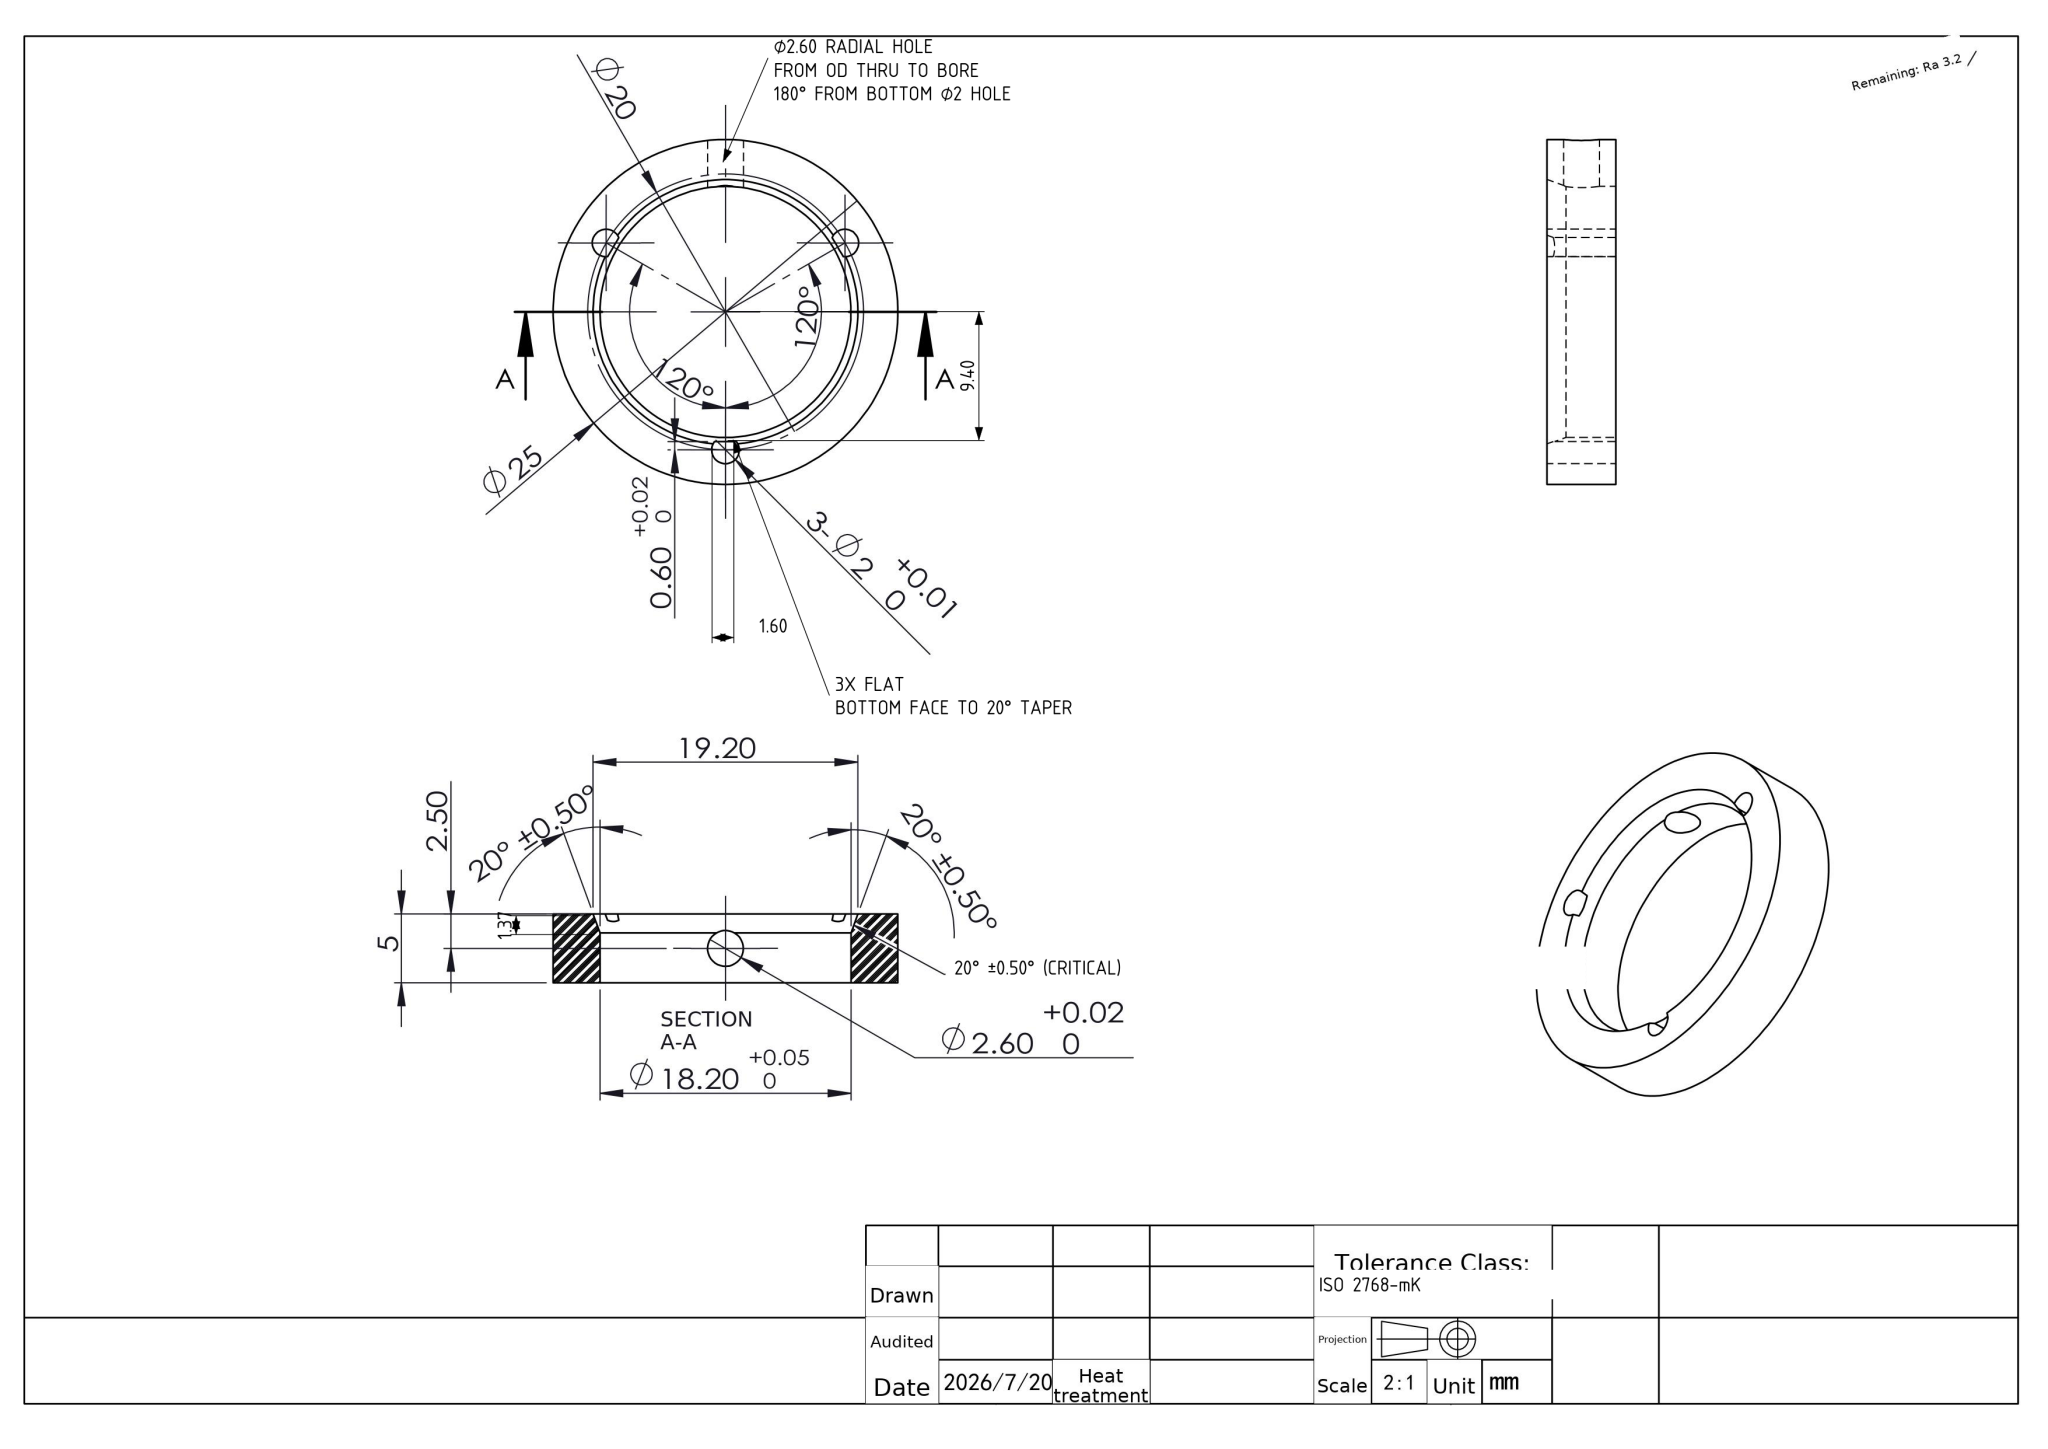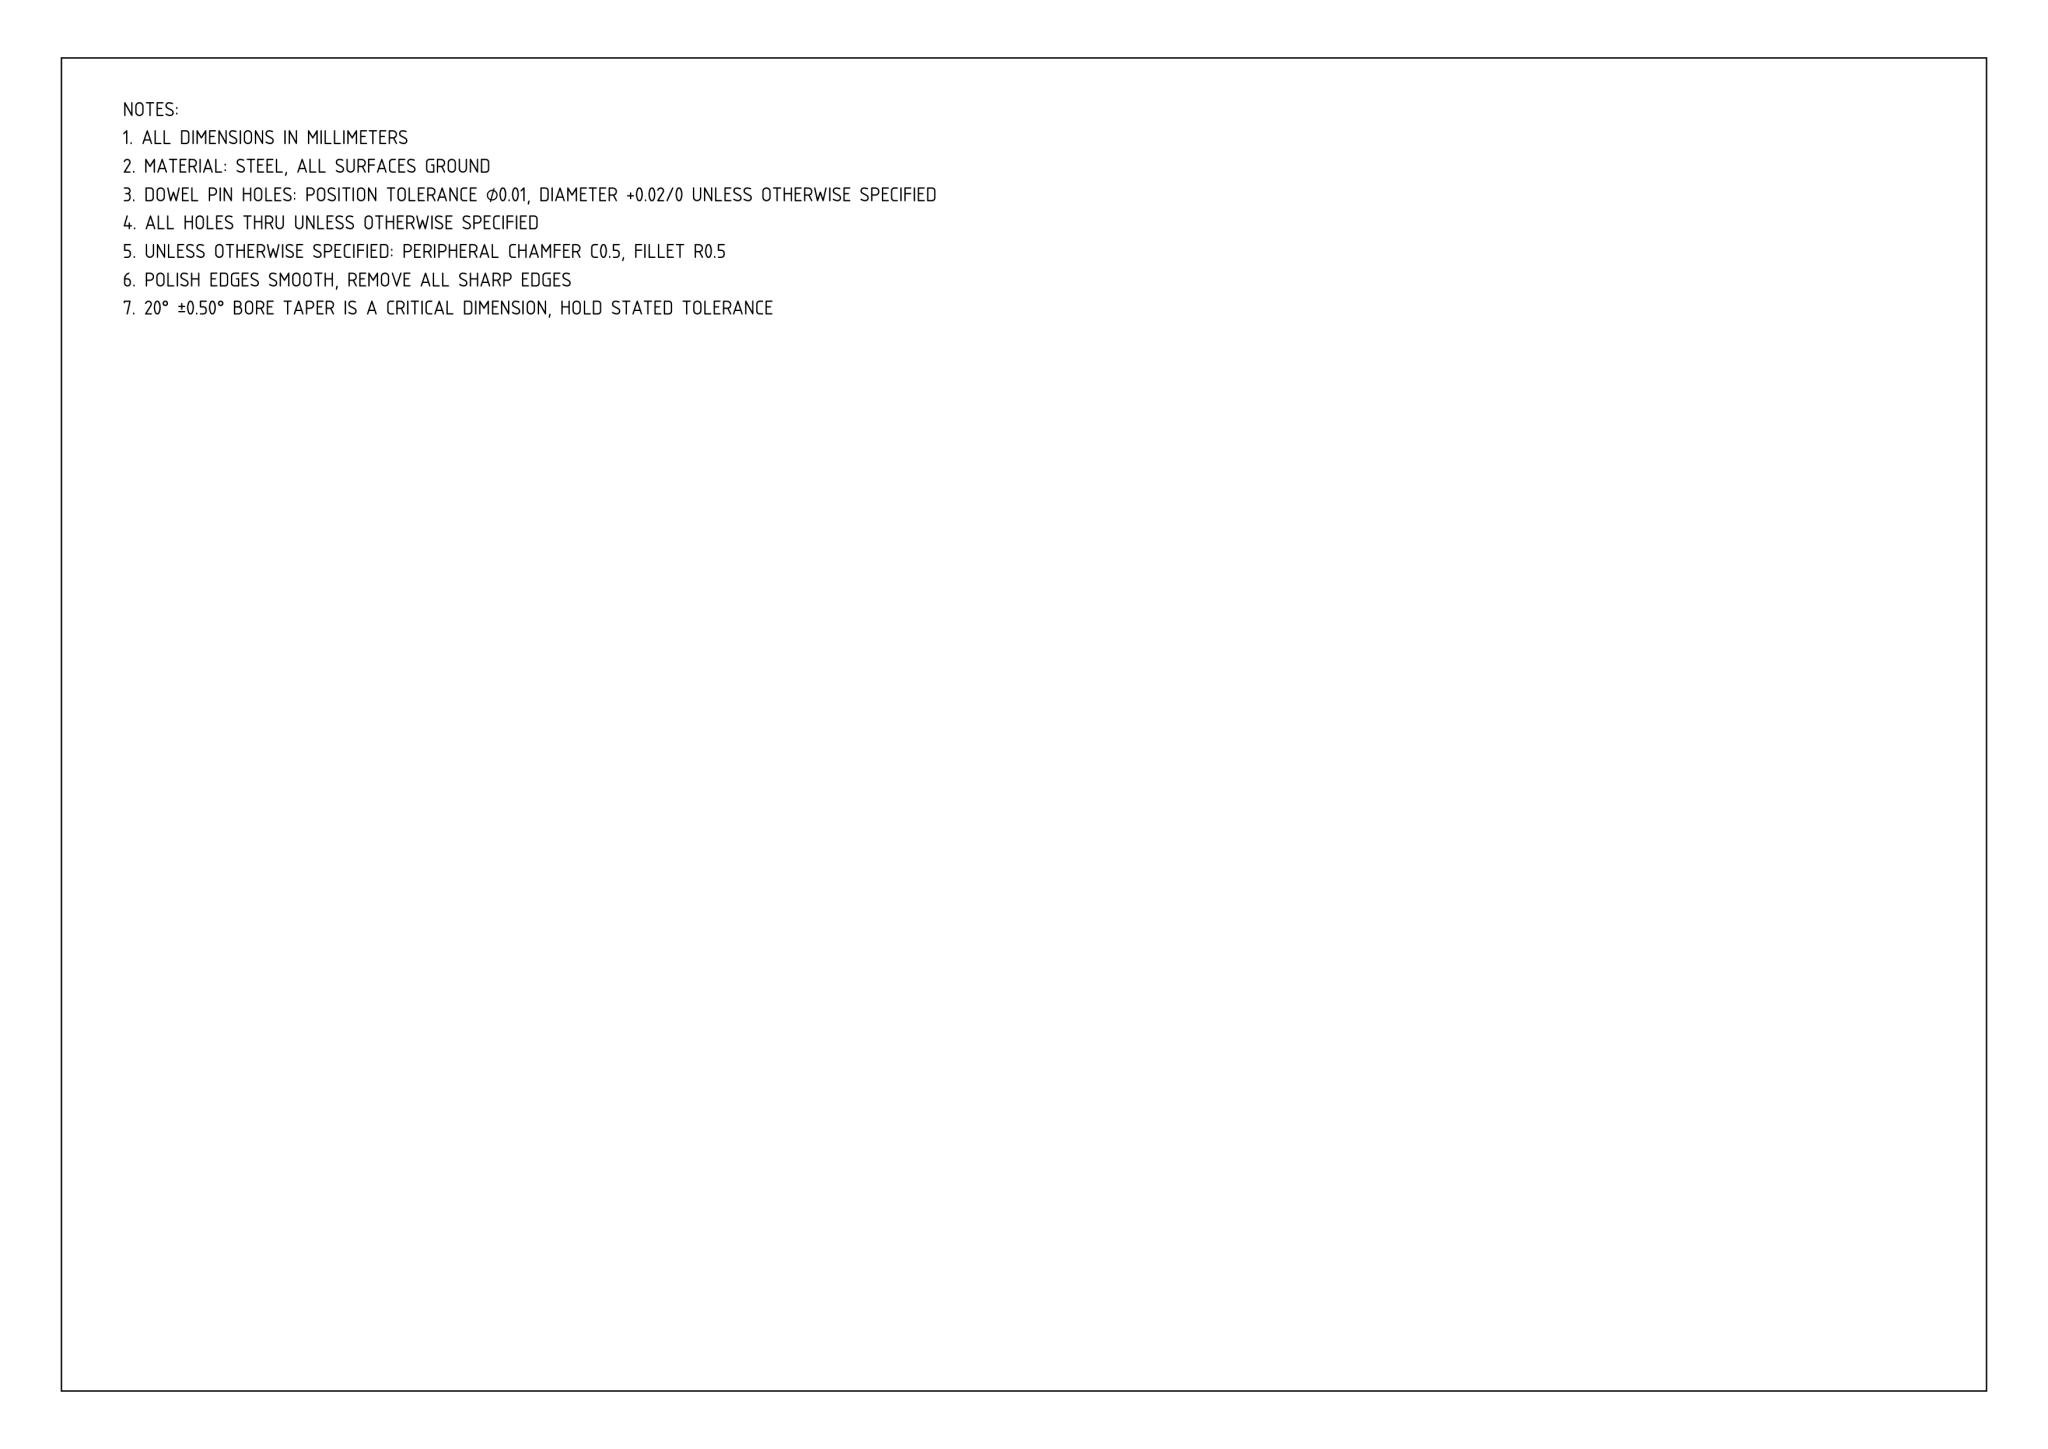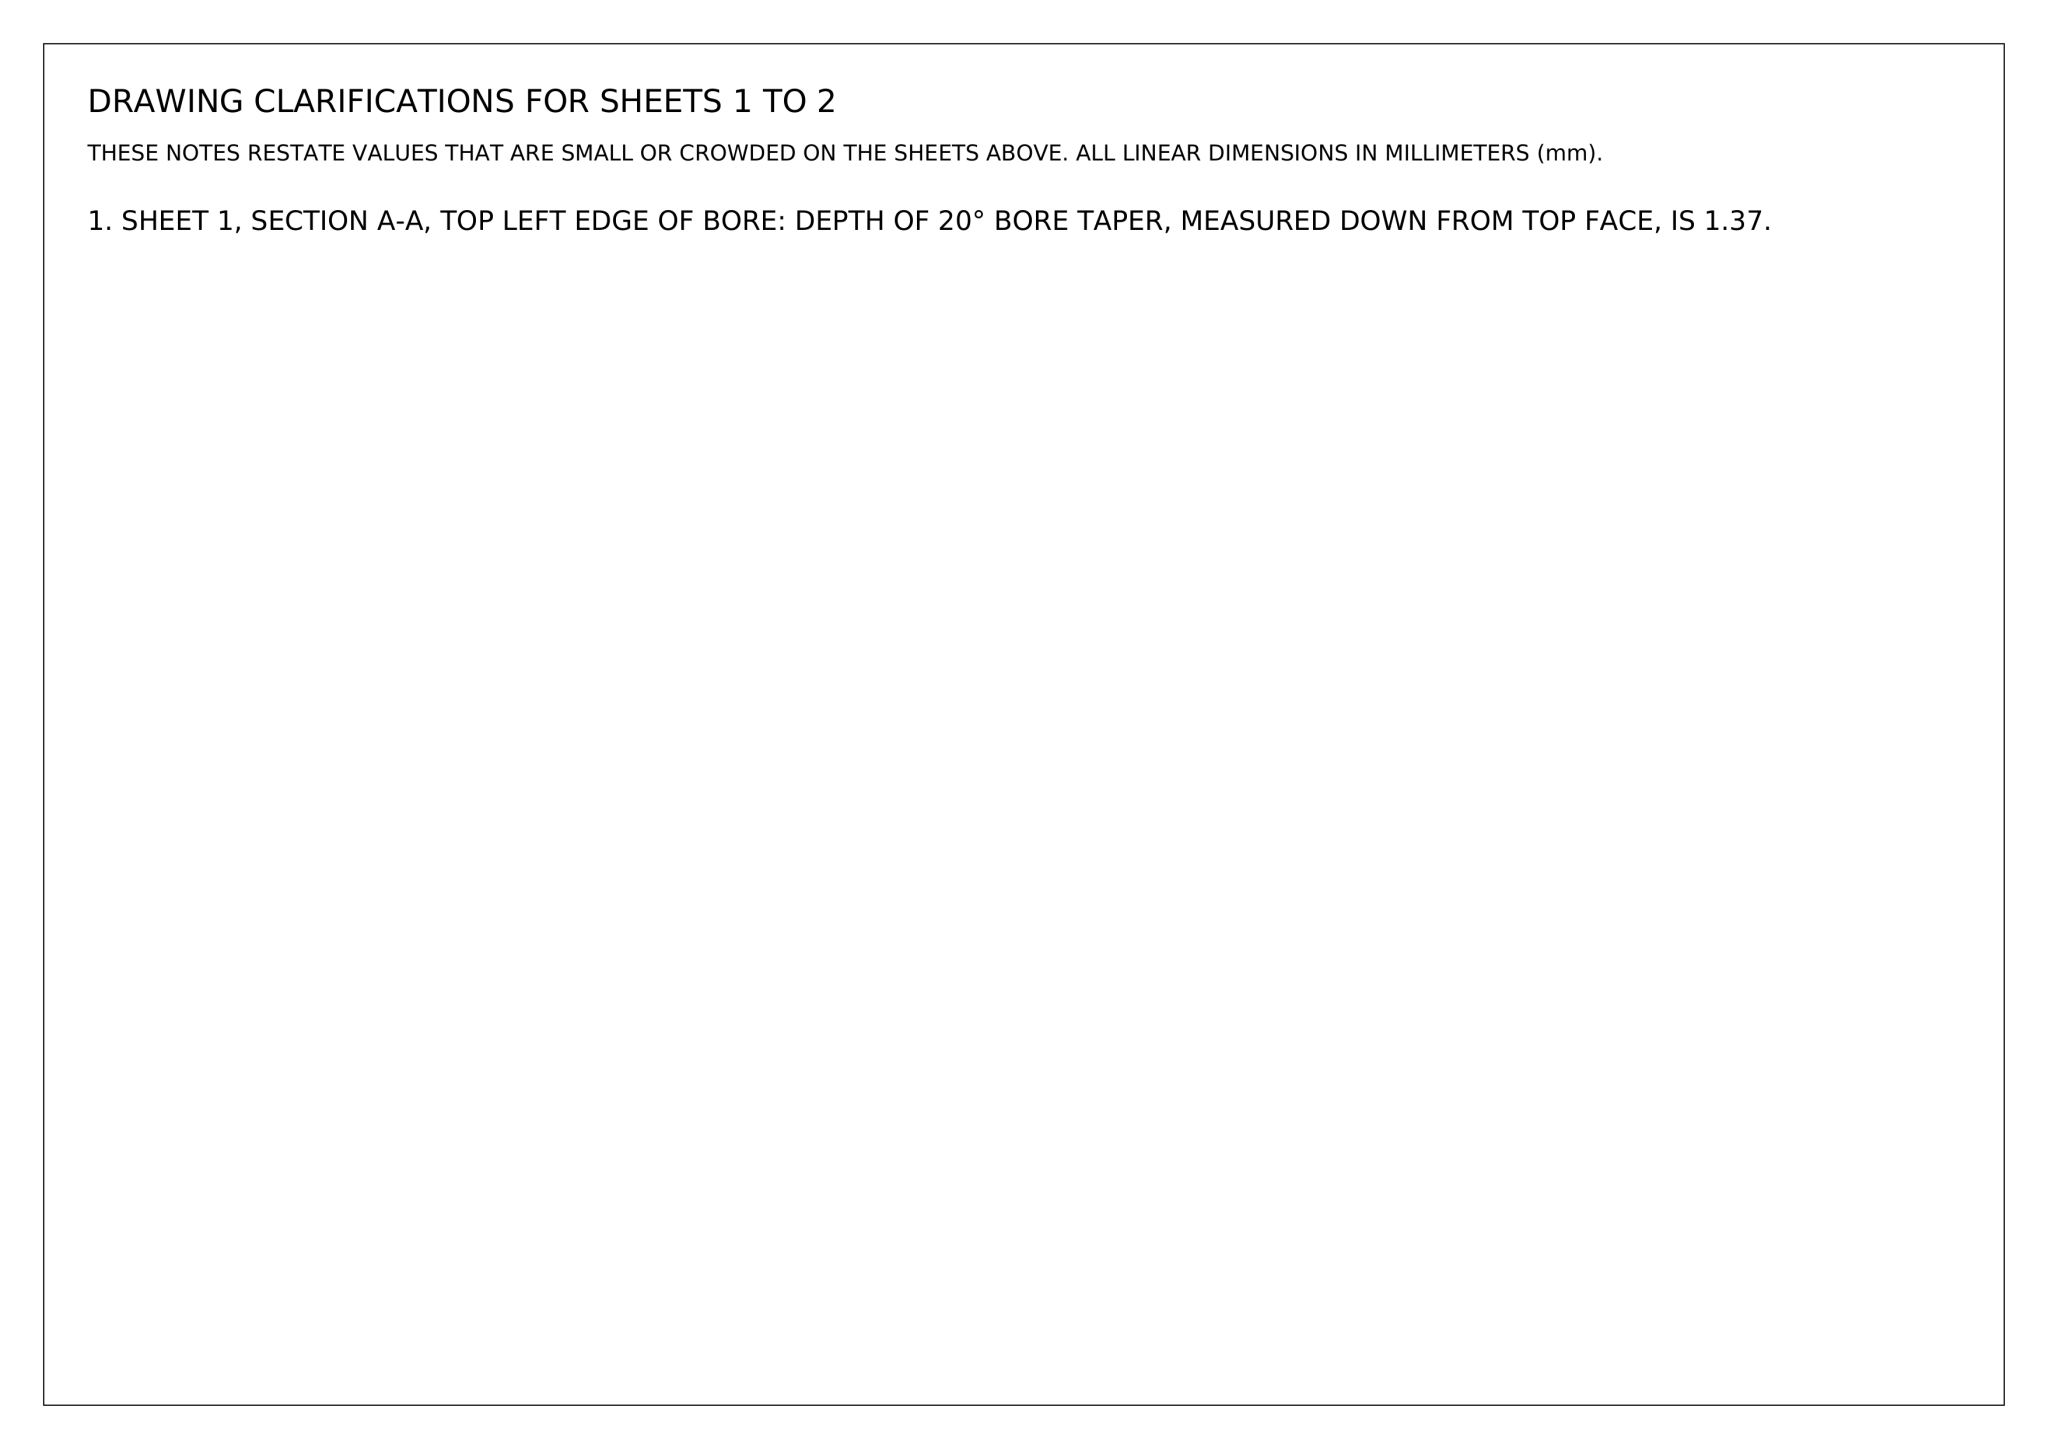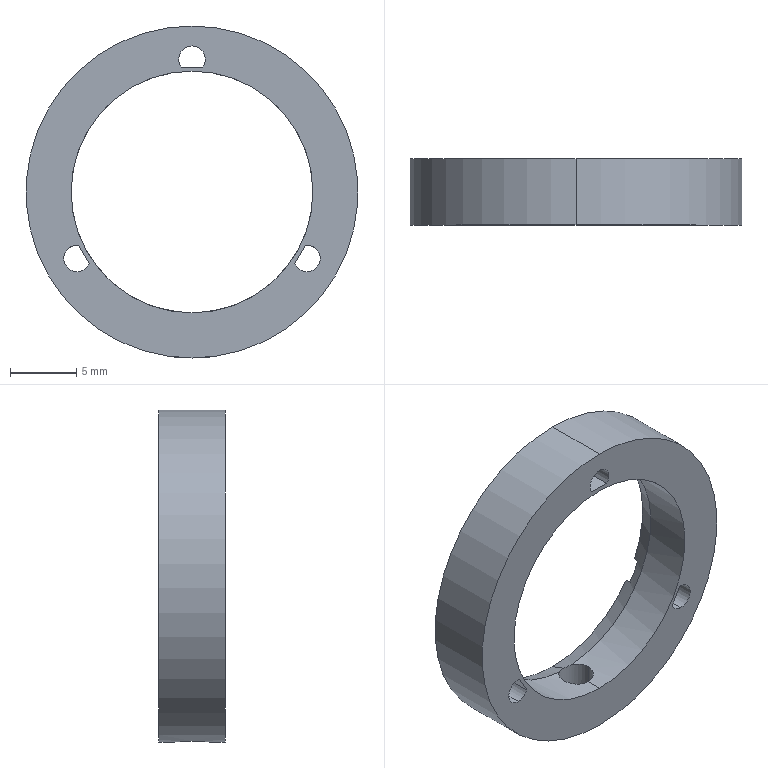Part | NX | mm | 1 solid | 21 faces | box 25 x 5 x 25 mm | volume 1075 mm3 | cylinder 14 | plane 5 | cone 2 | commonest cylinder face diameters 2 x8 2.6 x2 18.2 x2 25 x2